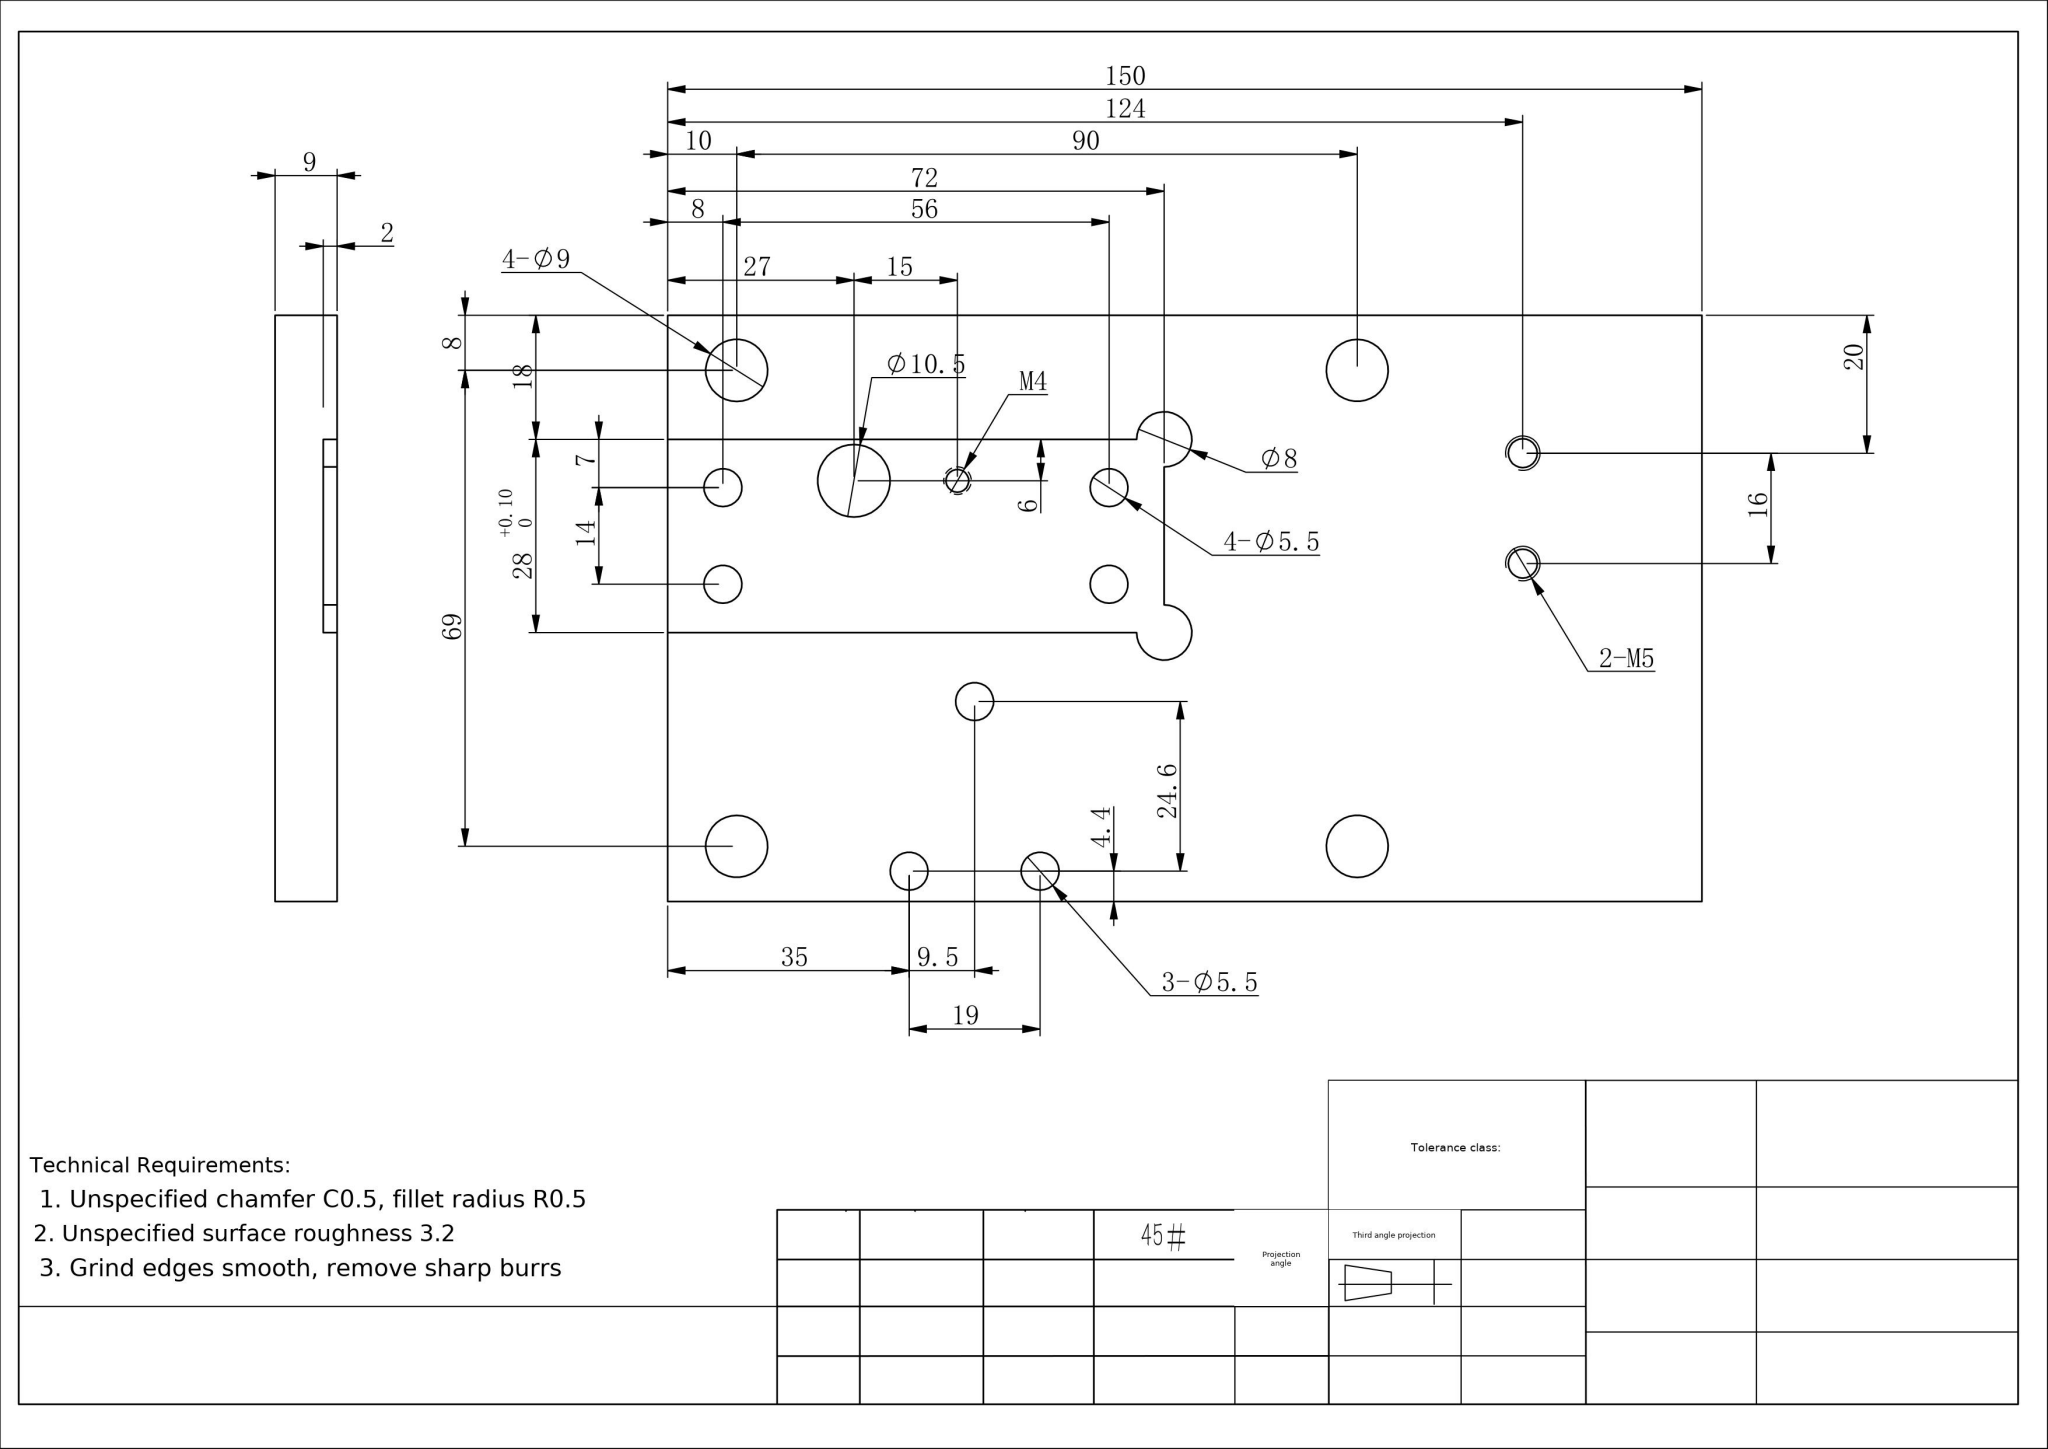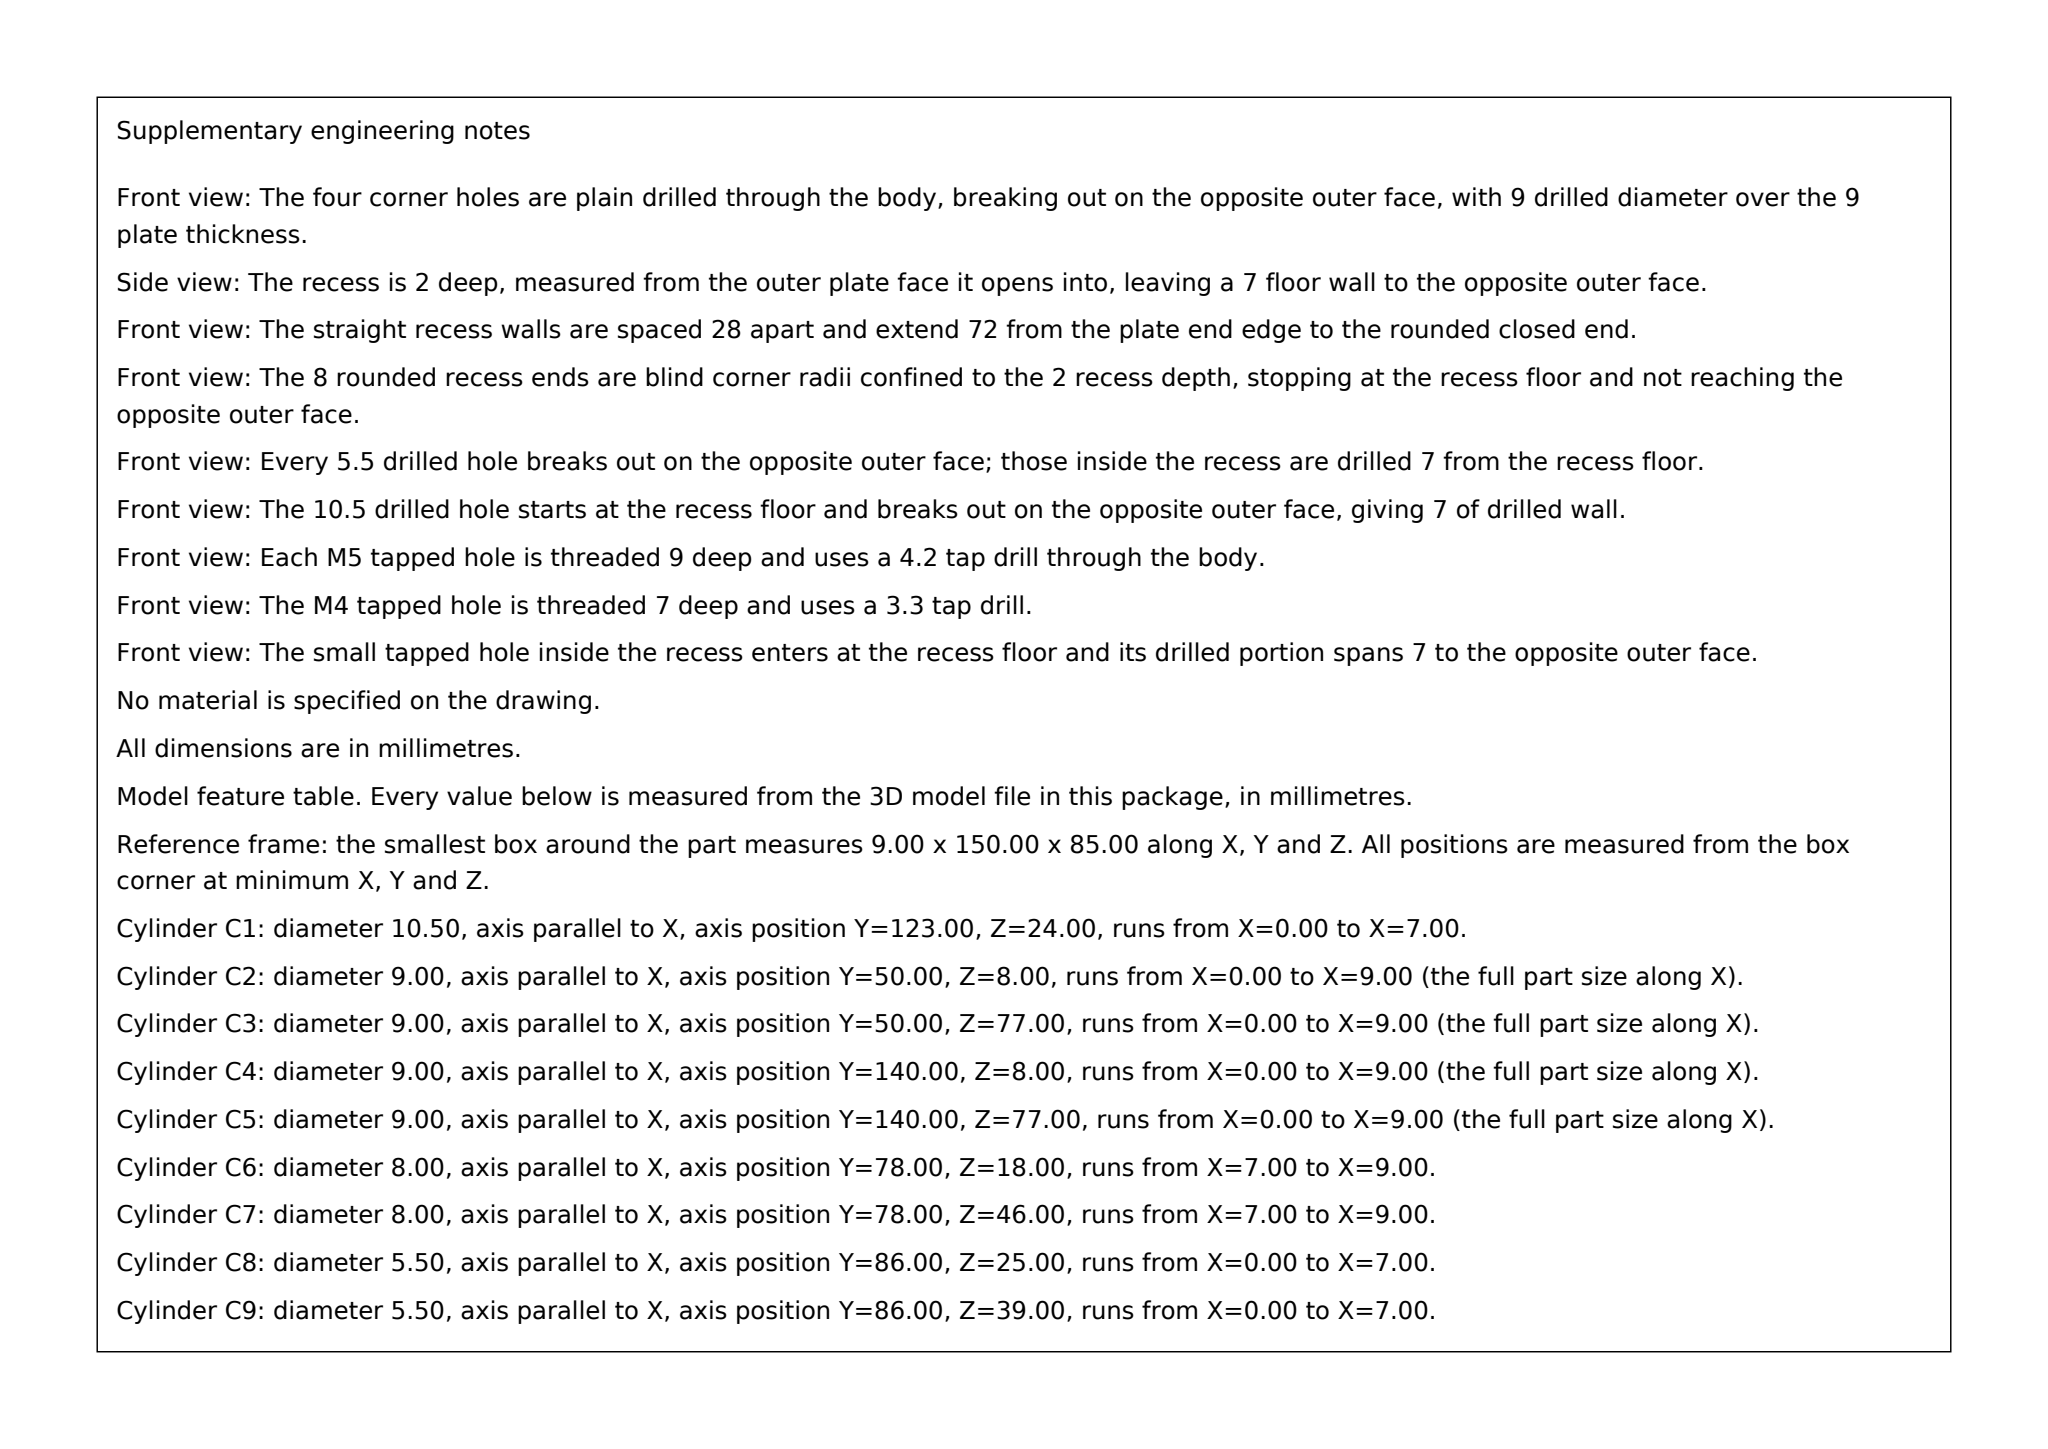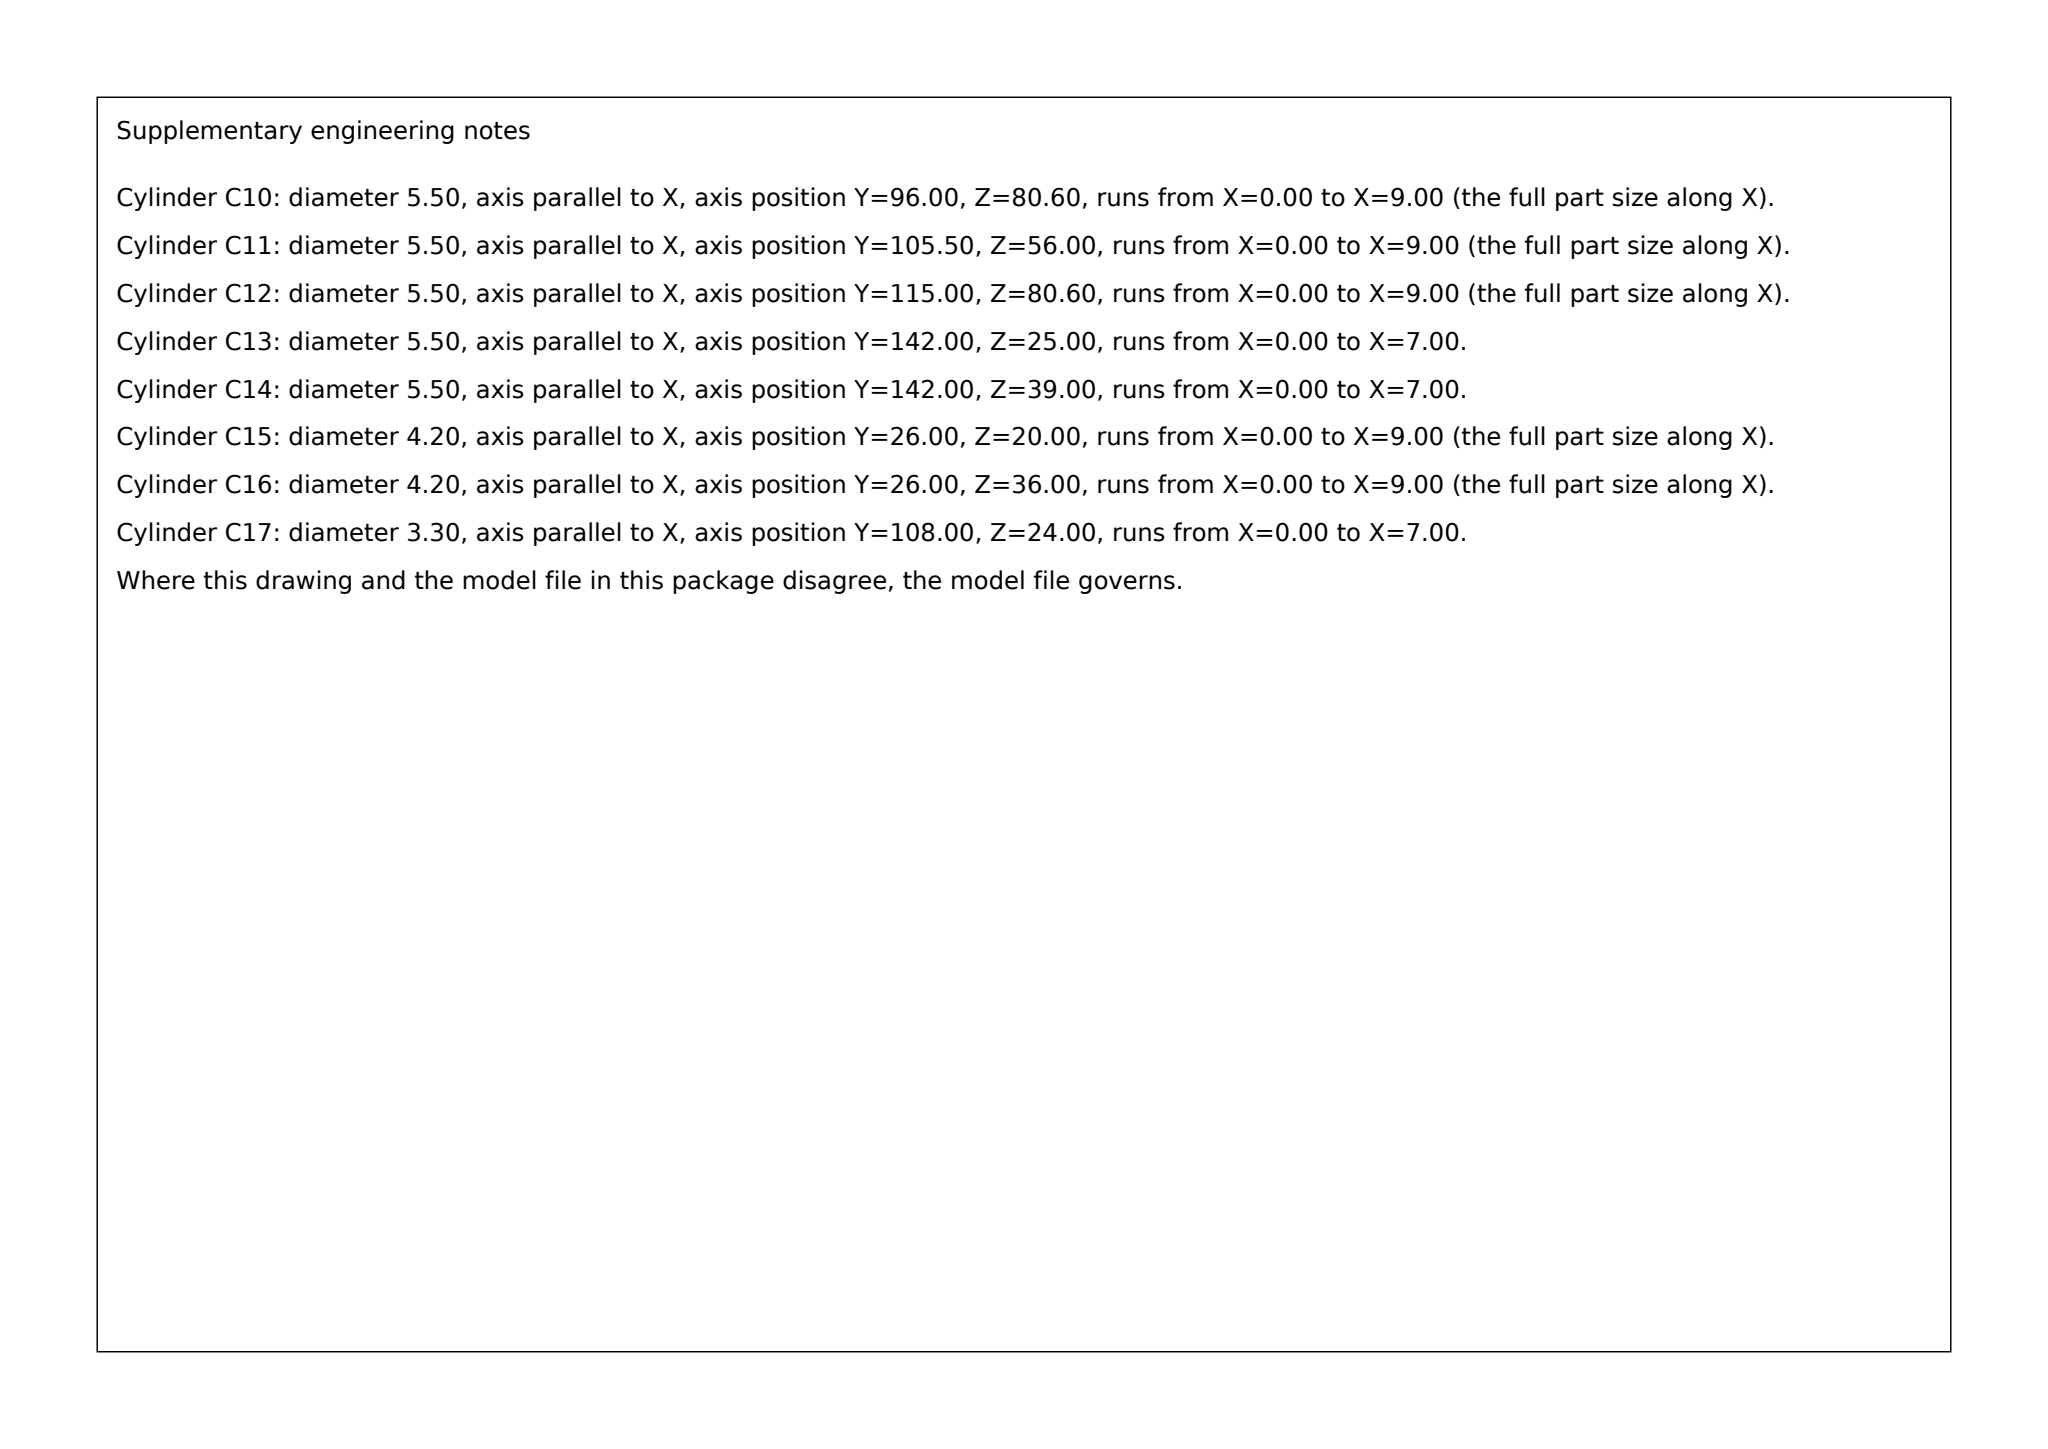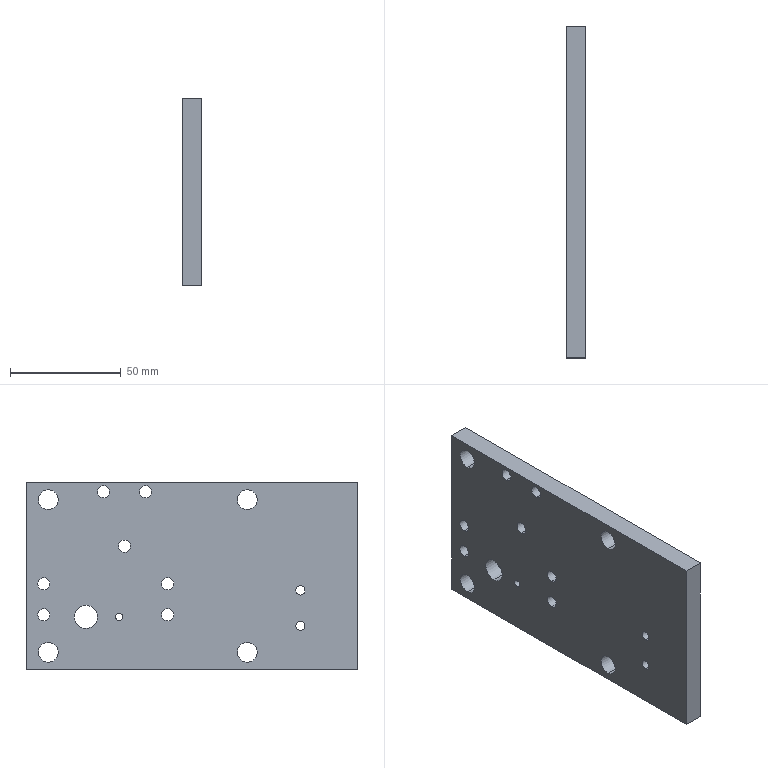Part | SolidWorks | mm | material 45# | 1 solid | 43 faces | box 9 x 150 x 85 mm | volume 106055 mm3 | cylinder 33 | plane 10 | commonest cylinder face diameters 5.5 x14 9 x8 4.2 x4 8 x3 3.3 x2 10.5 x2
Drawing notes:
OVERALL PLATE HT 85, TOP EDGE TO BOTTOM EDGE | from the solid: bbox_xyz z = 85.0; z planes at 0.0 and 85.0
TOL GRADE: X.X= ±0.02 | from the solid: Title block tolerance note; not derived from geometry
build123d program:
from build123d import *

# Parameters (mm, degrees)
SKETCH1_W                        = 85
SKETCH1_H                        = 150
BOSS_EXTRUDE1_DEPTH              = 9
SKETCH2_W                        = 28
SKETCH2_H                        = 72
CUT_EXTRUDE1_DEPTH               = 2
SKETCH3_R                        = 4
CUT_EXTRUDE2_DEPTH               = 2
SKETCH4_R                        = 4.5
CUT_EXTRUDE3_DEPTH               = 22
F_10_5_10_5_DIAMETER_HOLE1_D     = 10.5
F_10_5_10_5_DIAMETER_HOLE1_DEPTH = 30
F_10_5_10_5_DIAMETER_HOLE1_TIP   = 3.155
M5_TAPPED_HOLE1_D                = 4.2
M5_TAPPED_HOLE1_DEPTH            = 14
M5_TAPPED_HOLE1_TIP              = 1.262
F_5_5_5_5_DIAMETER_HOLE1_D       = 5.5
F_5_5_5_5_DIAMETER_HOLE1_DEPTH   = 30
F_5_5_5_5_DIAMETER_HOLE1_TIP     = 1.652
F_5_5_5_5_DIAMETER_HOLE2_D       = 5.5
F_5_5_5_5_DIAMETER_HOLE2_DEPTH   = 30
F_5_5_5_5_DIAMETER_HOLE2_TIP     = 1.652
M4_TAPPED_HOLE1_D                = 3.3
M4_TAPPED_HOLE1_DEPTH            = 11.5
M4_TAPPED_HOLE1_TIP              = 0.9914


with BuildPart() as part:
    # Sketch1 → Boss-Extrude1 (new body)
    with BuildSketch(Plane(origin=(0, 0, 0), x_dir=(0, 0, -1), z_dir=(1, 0, 0))):
        with Locations((42.5, 75)):
            Rectangle(SKETCH1_W, SKETCH1_H)
    extrude(amount=BOSS_EXTRUDE1_DEPTH)

    # Sketch2 → Cut-Extrude1 (cut)
    with BuildSketch(Plane(origin=(9, 0, 0), x_dir=(0, 0, -1), z_dir=(1, 0, 0))):
        with Locations((53, 114)):
            Rectangle(SKETCH2_W, SKETCH2_H)
    extrude(amount=-CUT_EXTRUDE1_DEPTH, mode=Mode.SUBTRACT)

    # Sketch3 → Cut-Extrude2 (cut)
    with BuildSketch(Plane(origin=(9, 0, 0), x_dir=(0, 0, -1), z_dir=(1, 0, 0))):
        with Locations((67, 78)):
            Circle(SKETCH3_R)
        with Locations((39, 78)):
            Circle(SKETCH3_R)
    extrude(amount=-CUT_EXTRUDE2_DEPTH, mode=Mode.SUBTRACT)

    # Sketch4 → Cut-Extrude3 (cut)
    with BuildSketch(Plane(origin=(9, 0, 0), x_dir=(0, 0, -1), z_dir=(1, 0, 0))):
        with Locations((8, 140)):
            Circle(SKETCH4_R)
        with Locations(Location((77, 140, 0), (0, 0, 180))):
            Circle(SKETCH4_R)
        with Locations((77, 50)):
            Circle(SKETCH4_R)
        with Locations(Location((8, 50, 0), (0, 0, 180))):
            Circle(SKETCH4_R)
    extrude(amount=-CUT_EXTRUDE3_DEPTH, mode=Mode.SUBTRACT)

    # 10.5 _10.5_ Diameter Hole1
    with Locations(Plane(origin=(7, 0, 0), x_dir=(0, 0, -1), z_dir=(1, 0, 0))):
        with Locations((61, 123)):
            Hole(F_10_5_10_5_DIAMETER_HOLE1_D / 2, depth=F_10_5_10_5_DIAMETER_HOLE1_DEPTH)
            with Locations((0, 0, -(F_10_5_10_5_DIAMETER_HOLE1_DEPTH + F_10_5_10_5_DIAMETER_HOLE1_TIP / 2))):  # 118° drill point
                Cone(0, F_10_5_10_5_DIAMETER_HOLE1_D / 2, F_10_5_10_5_DIAMETER_HOLE1_TIP, mode=Mode.SUBTRACT)

    # M5 Tapped Hole1
    with Locations(Plane(origin=(9, 0, 0), x_dir=(0, 0, -1), z_dir=(1, 0, 0))):
        with Locations((49, 26), (65, 26)):
            Hole(M5_TAPPED_HOLE1_D / 2, depth=M5_TAPPED_HOLE1_DEPTH)
            with Locations((0, 0, -(M5_TAPPED_HOLE1_DEPTH + M5_TAPPED_HOLE1_TIP / 2))):  # 118° drill point
                Cone(0, M5_TAPPED_HOLE1_D / 2, M5_TAPPED_HOLE1_TIP, mode=Mode.SUBTRACT)

    # 5.5 _5.5_ Diameter Hole1
    with Locations(Plane.ZY):
        with Locations((-60, 142), (-46, 142), (-60, 86), (-46, 86)):
            Hole(F_5_5_5_5_DIAMETER_HOLE1_D / 2, depth=F_5_5_5_5_DIAMETER_HOLE1_DEPTH)
            with Locations((0, 0, -(F_5_5_5_5_DIAMETER_HOLE1_DEPTH + F_5_5_5_5_DIAMETER_HOLE1_TIP / 2))):  # 118° drill point
                Cone(0, F_5_5_5_5_DIAMETER_HOLE1_D / 2, F_5_5_5_5_DIAMETER_HOLE1_TIP, mode=Mode.SUBTRACT)

    # 5.5 _5.5_ Diameter Hole2
    with Locations(Plane.ZY):
        with Locations((-29, 105.5), (-4.403, 115), (-4.403, 96)):
            Hole(F_5_5_5_5_DIAMETER_HOLE2_D / 2, depth=F_5_5_5_5_DIAMETER_HOLE2_DEPTH)
            with Locations((0, 0, -(F_5_5_5_5_DIAMETER_HOLE2_DEPTH + F_5_5_5_5_DIAMETER_HOLE2_TIP / 2))):  # 118° drill point
                Cone(0, F_5_5_5_5_DIAMETER_HOLE2_D / 2, F_5_5_5_5_DIAMETER_HOLE2_TIP, mode=Mode.SUBTRACT)

    # M4 Tapped Hole1
    with Locations(Plane.ZY):
        with Locations((-61, 108)):
            Hole(M4_TAPPED_HOLE1_D / 2, depth=M4_TAPPED_HOLE1_DEPTH)
            with Locations((0, 0, -(M4_TAPPED_HOLE1_DEPTH + M4_TAPPED_HOLE1_TIP / 2))):  # 118° drill point
                Cone(0, M4_TAPPED_HOLE1_D / 2, M4_TAPPED_HOLE1_TIP, mode=Mode.SUBTRACT)


solid = part.part